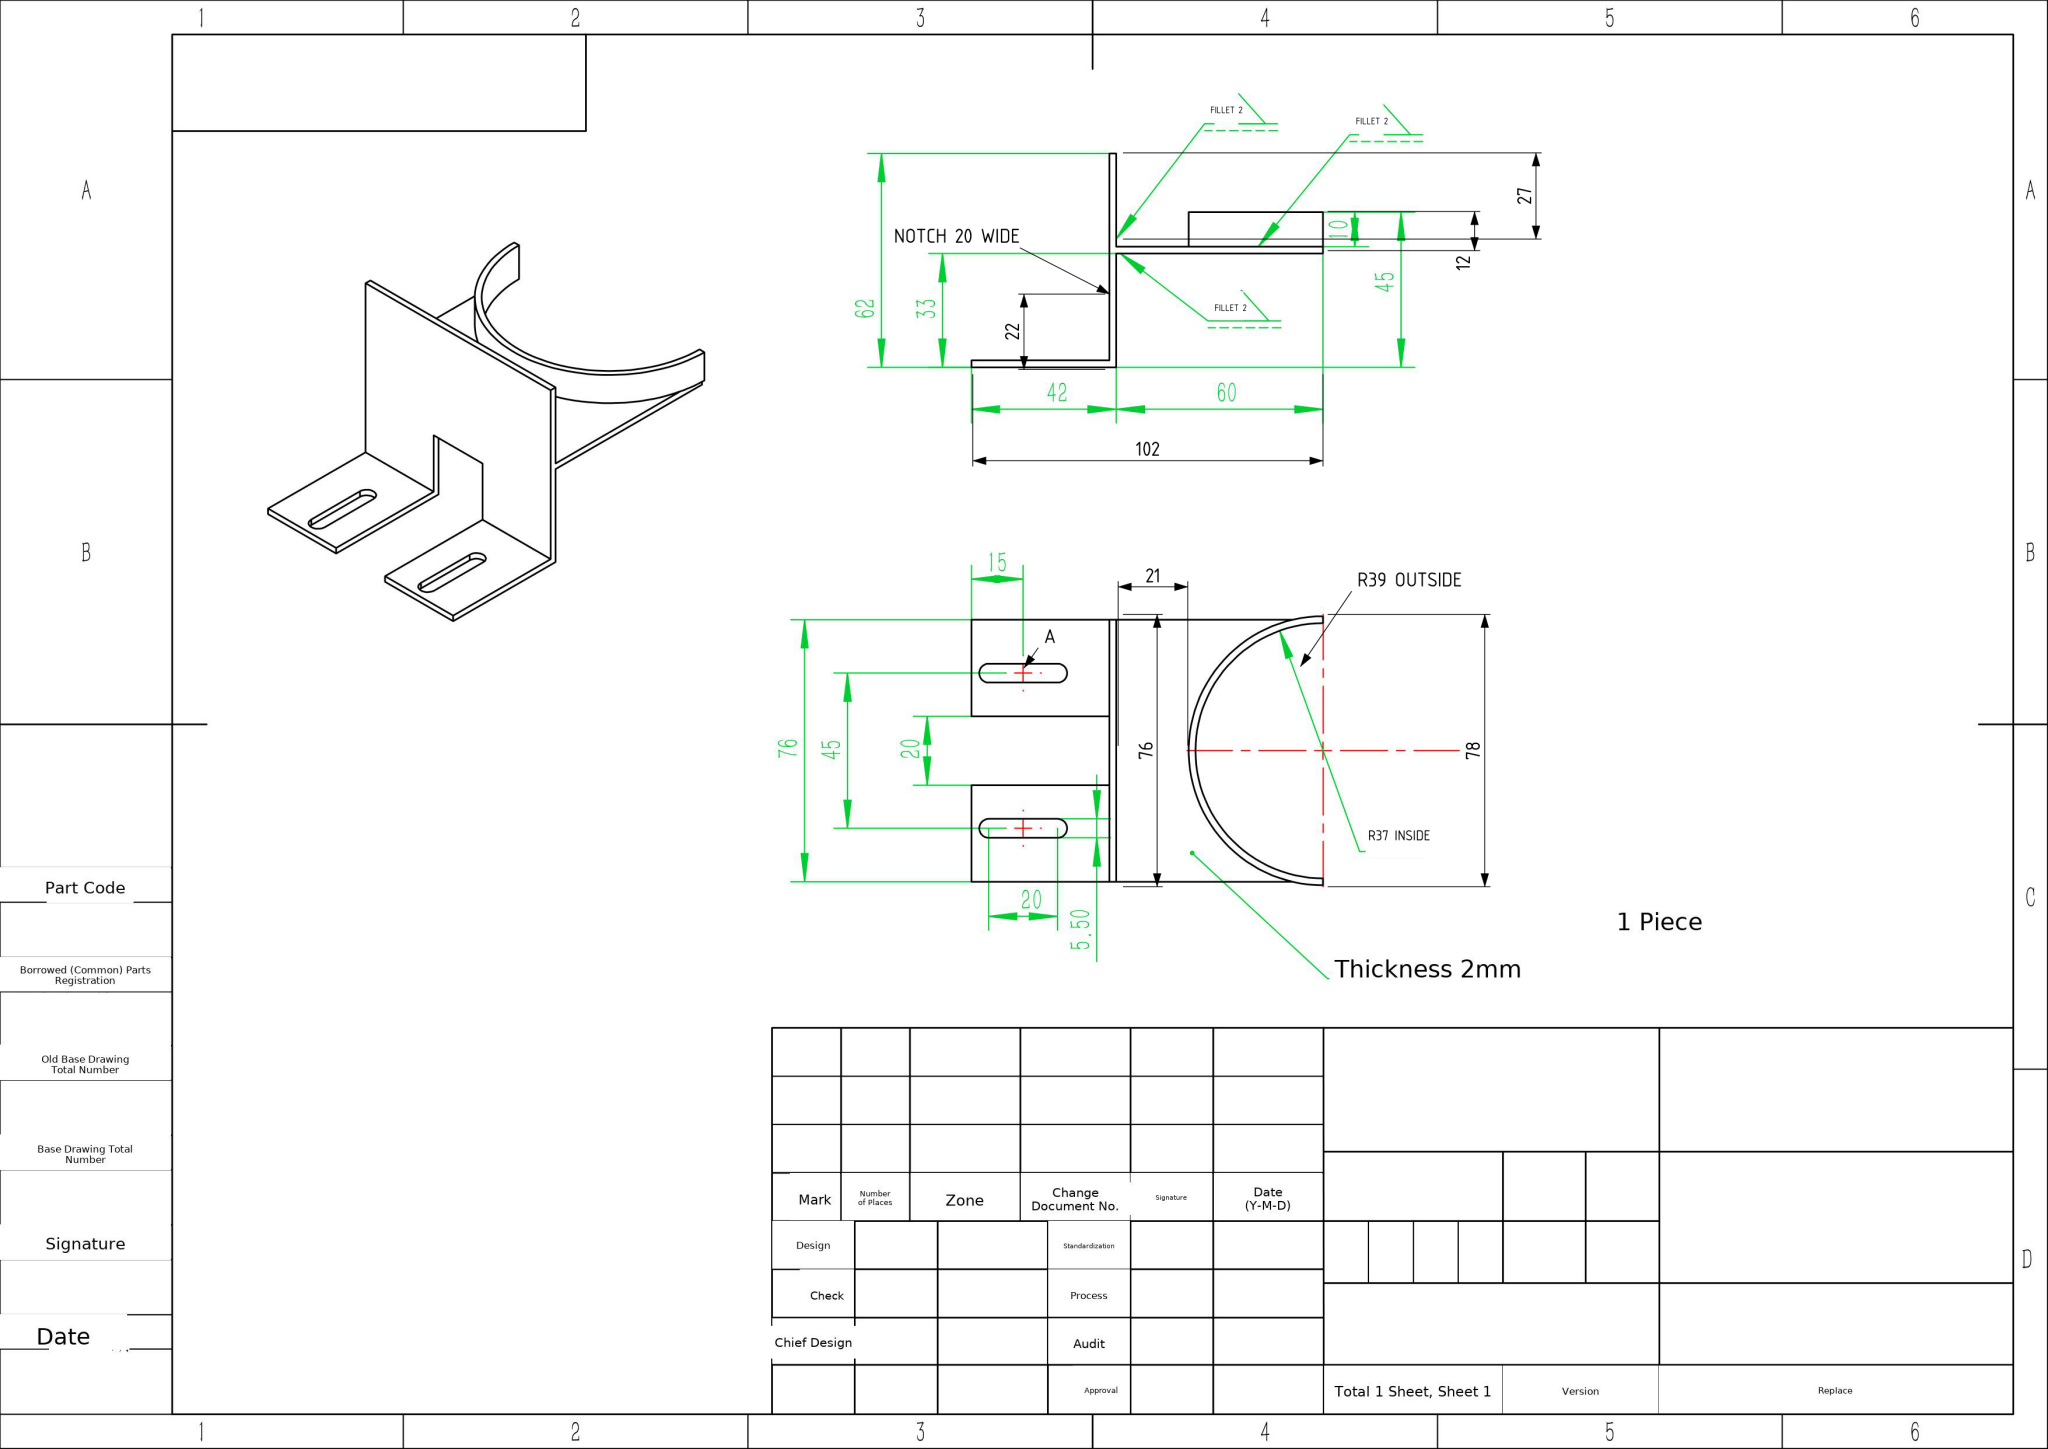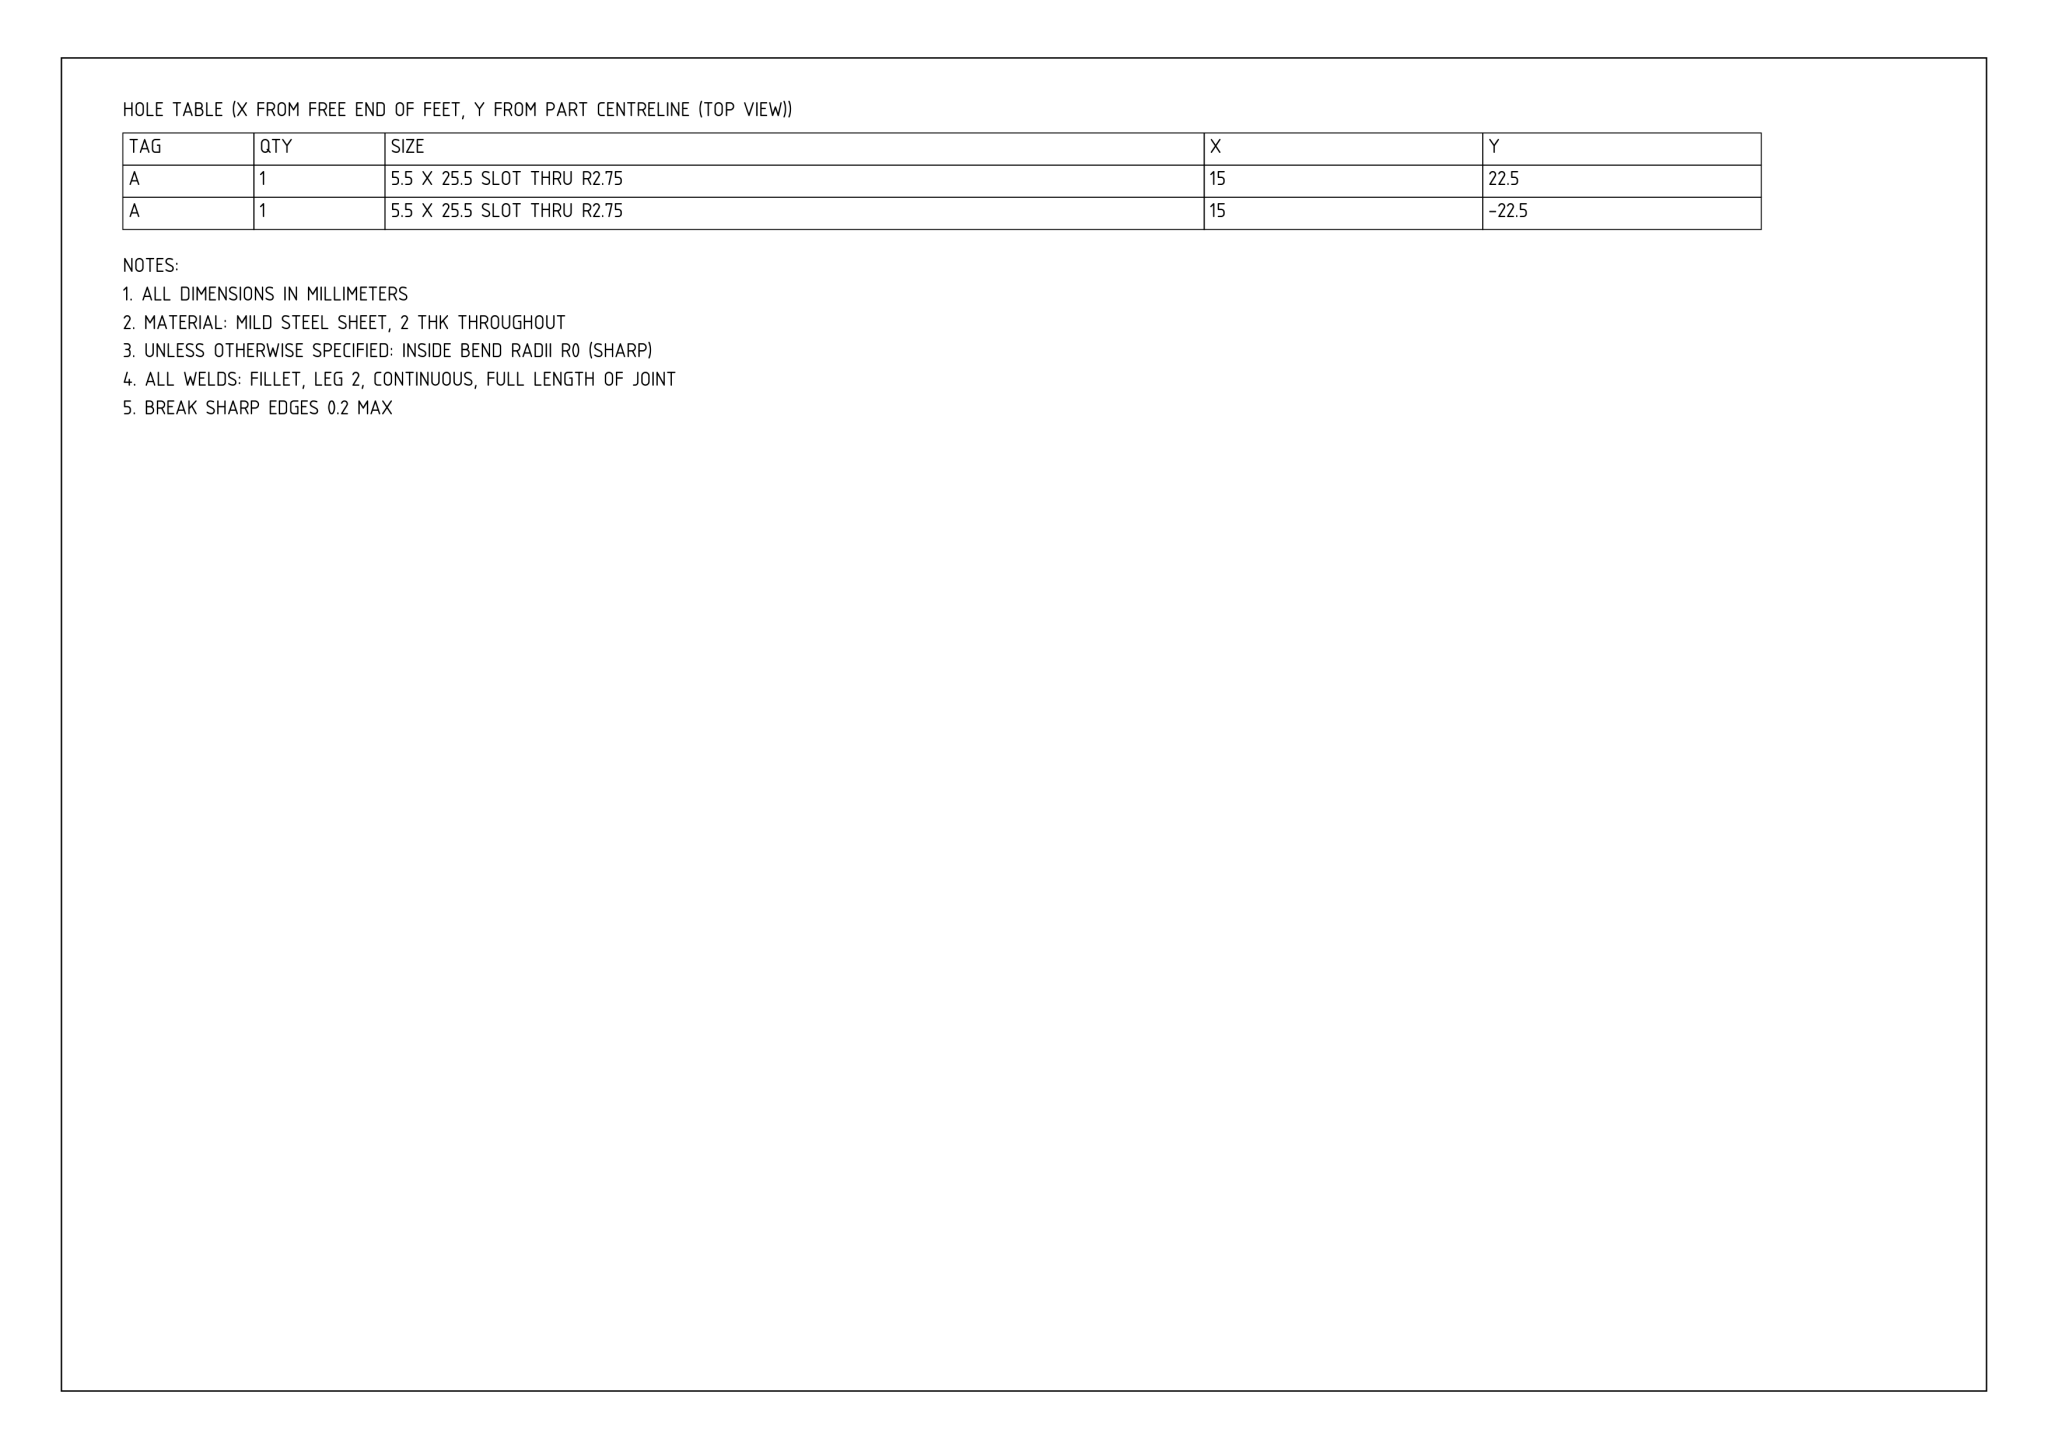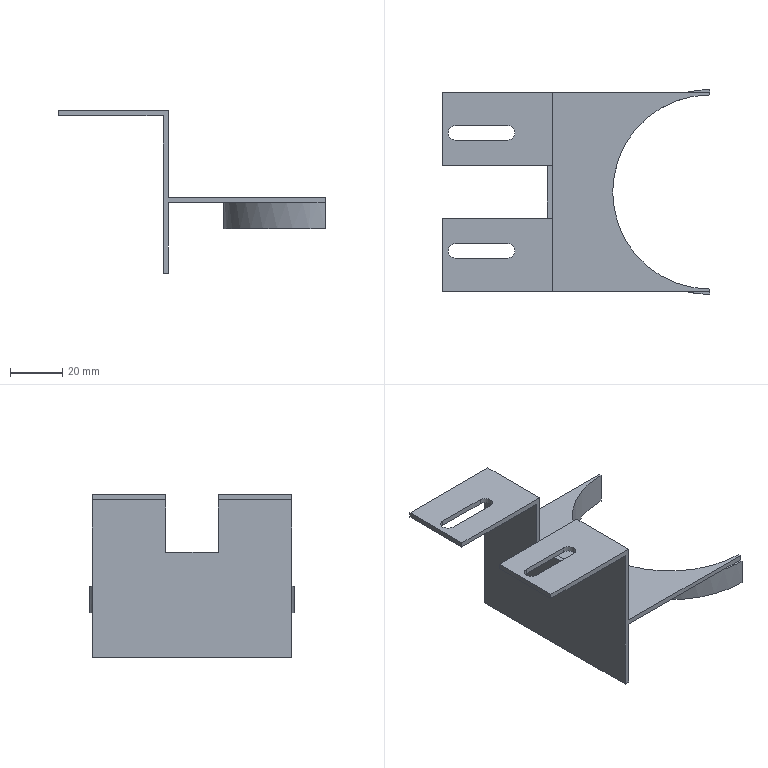Part | NX | mm | 1 solid | 34 faces | box 102 x 78 x 62 mm | volume 19696 mm3 | plane 26 | cylinder 8 | commonest cylinder face diameters 5.5 x6 74 x1 78 x1